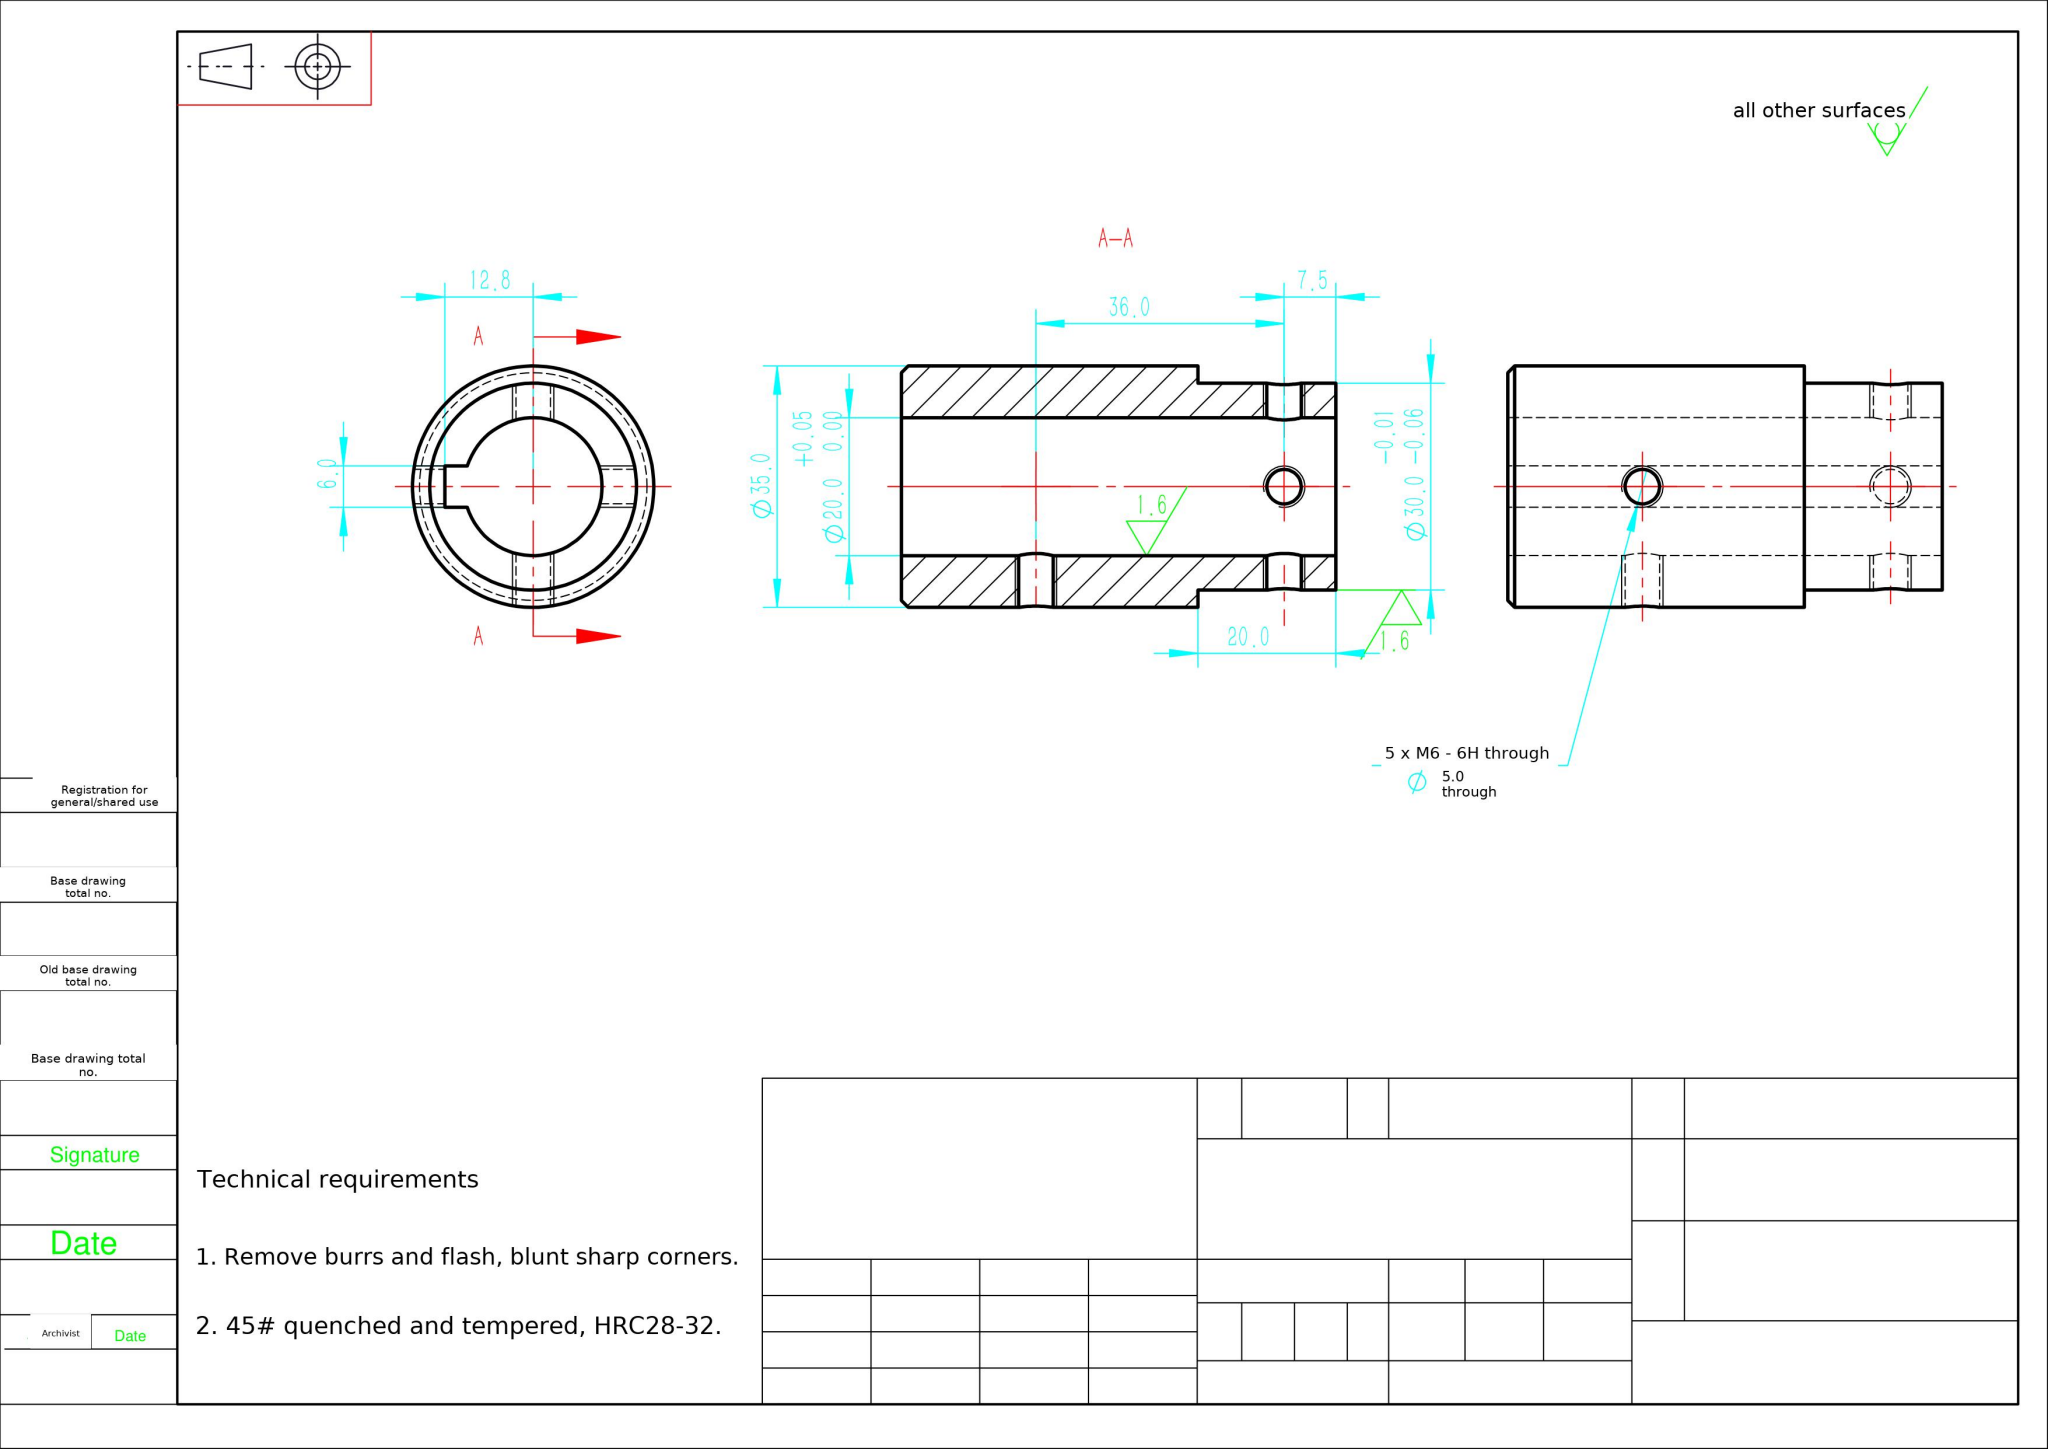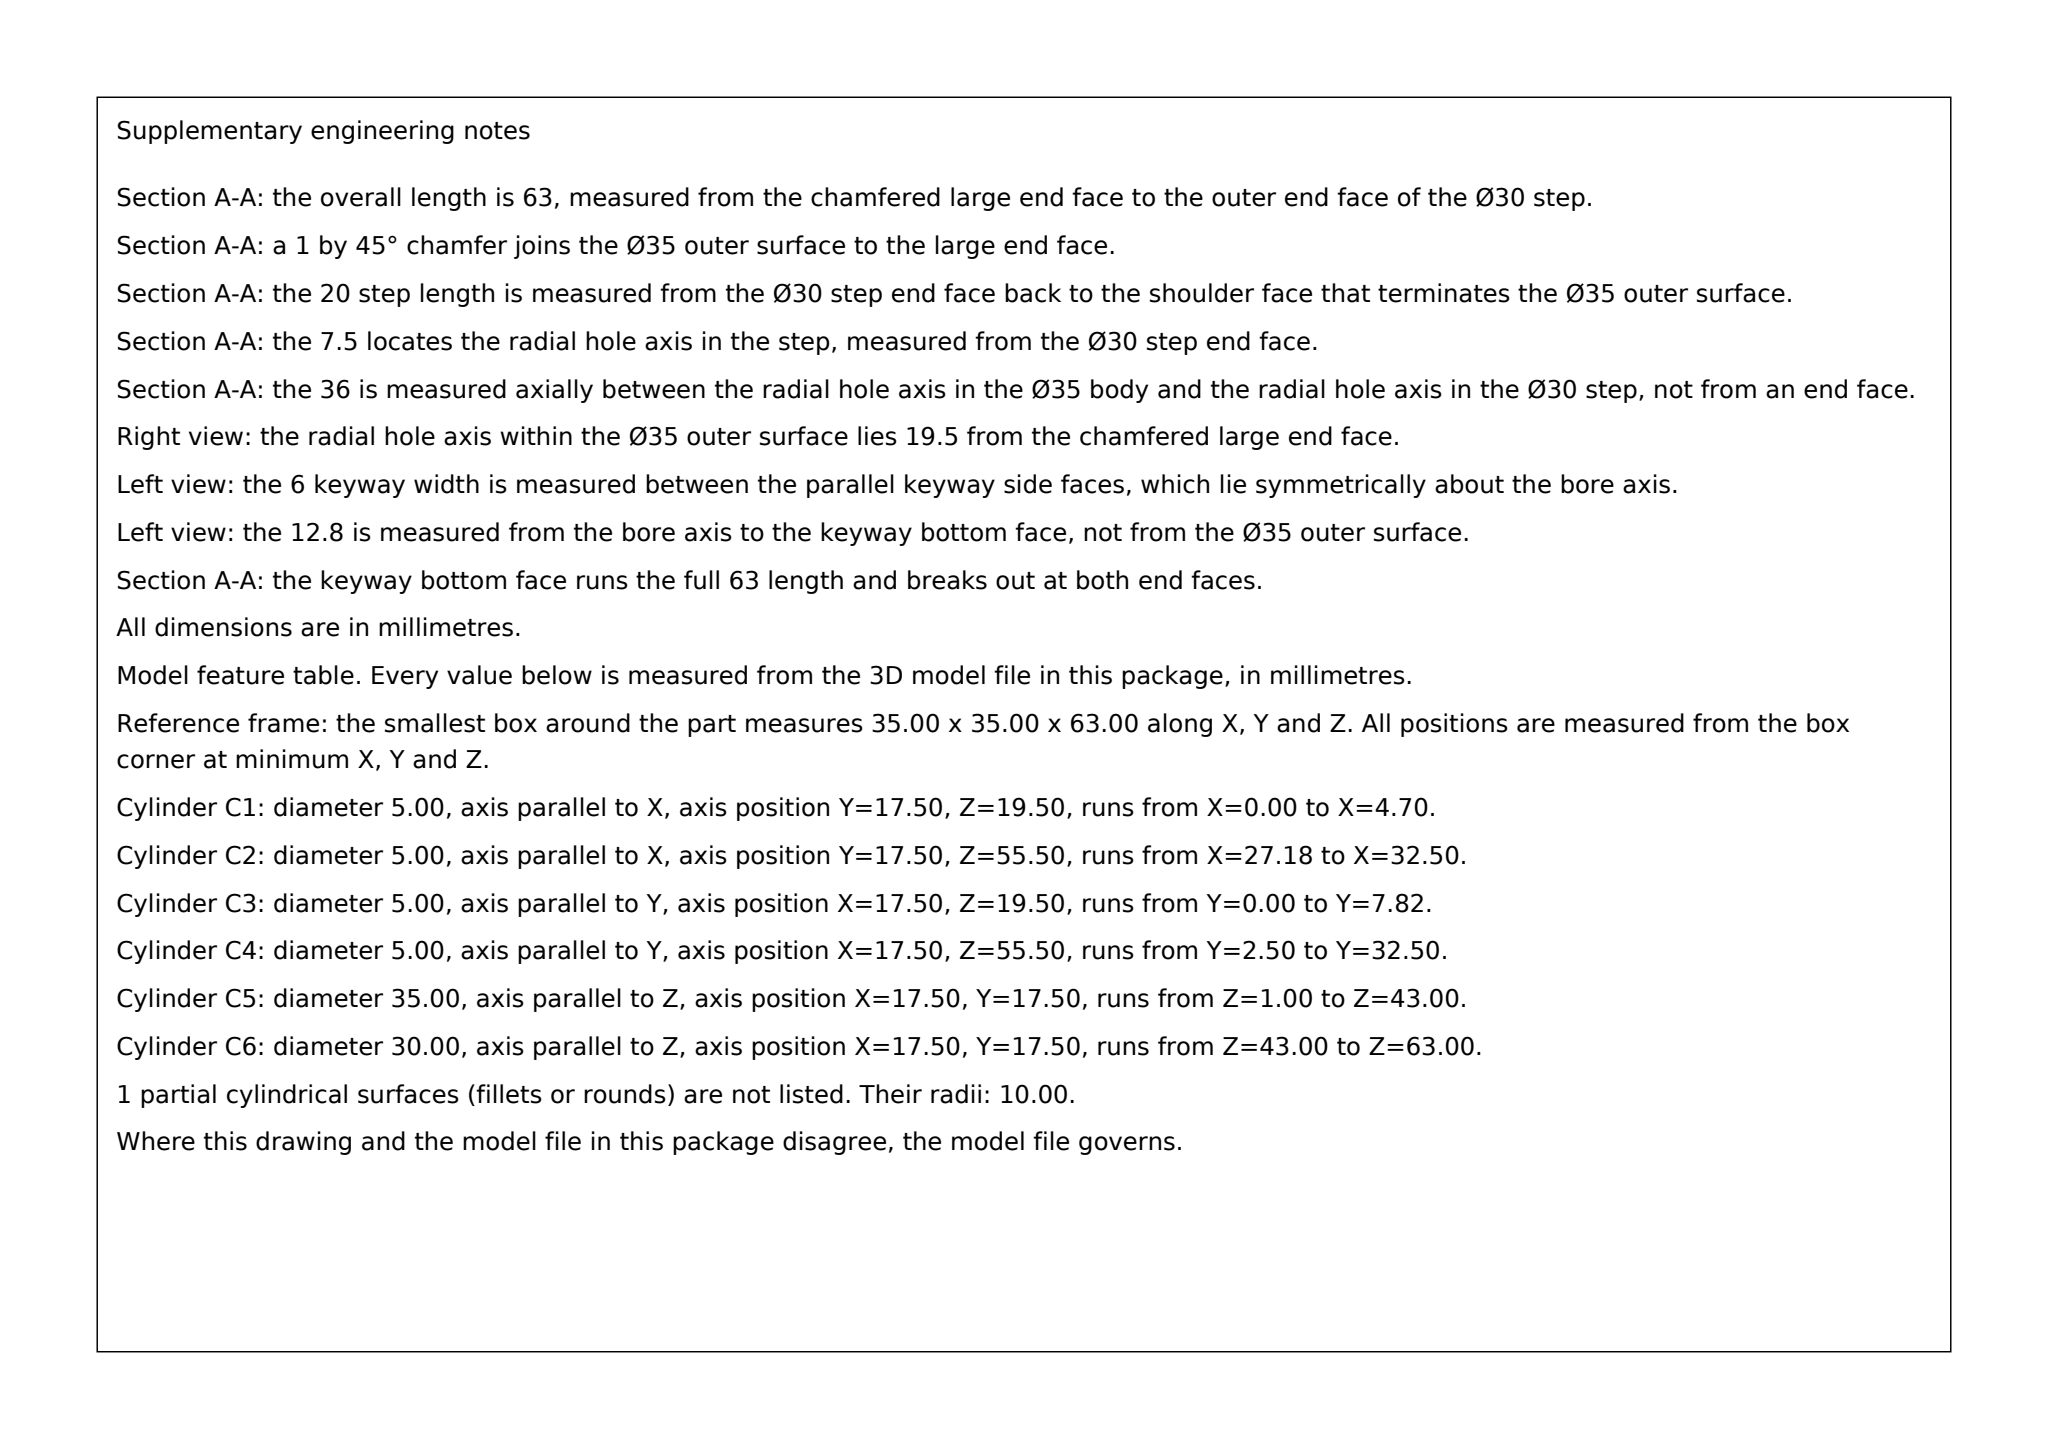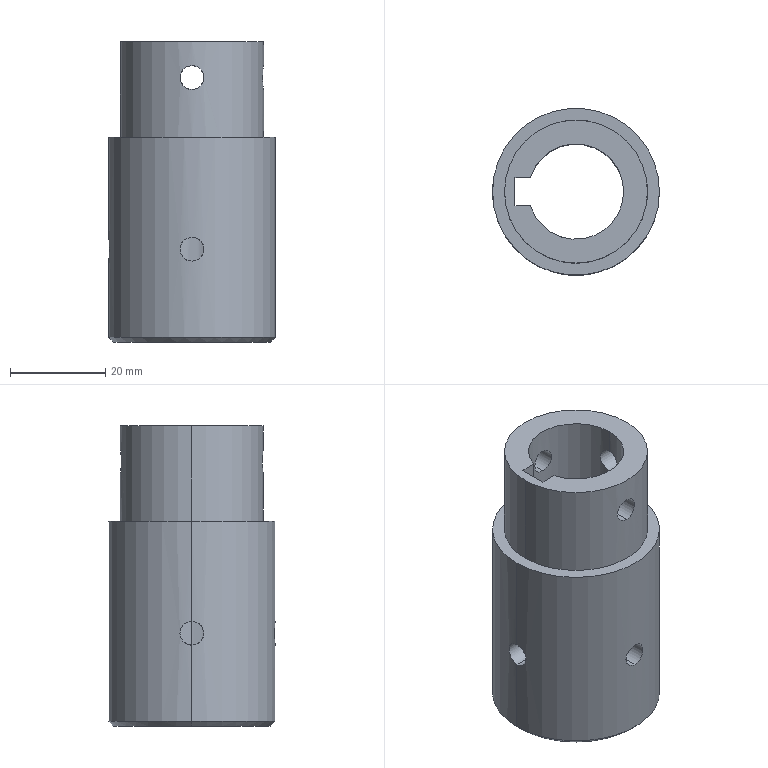Part | SolidWorks | mm | 1 solid | 24 faces | box 35 x 35 x 63 mm | volume 34011 mm3 | cylinder 16 | plane 6 | cone 2 | commonest cylinder face diameters 5 x10 30 x2 20 x2 35 x2
Drawing notes:
M6 HOLE 19.5 FM LH END ON KEYWAY CL, BREAKS INTO KEYWAY | from the solid: Ø5 cyl axis x at y=17.5, z=19.5, len 4.7 ending at keyway floor plane x=4.7 (keyway y 14.5/20.5)
M6 HOLE 19.5 FM LH END AT 90 DEG TO KEYWAY CL, 1 SIDE ONLY | from the solid: Ø5 cyl axis y at x=17.5, z=19.5, len 7.82 (Ø35 wall), single hole
2X M6 IN Ø30 BOSS 7.5 FM RH END AT 90 & 270 DEG TO KEYWAY CL | from the solid: Ø5 cyl axis y at x=17.5, z=55.5, len 5.32, count 4 faces = diametral pair in Ø30 boss (z 43-63)
M6 IN Ø30 BOSS 7.5 FM RH END IN KEYWAY CL PLANE, 90 DEG FM PAIR | from the solid: Ø5 cyl axis x at y=17.5, z=55.5, len 5.32, perpendicular to the y-axis pair at same station
5X M6 HOLES NOT EQSP - SEE ANGULAR NOTES, AXIAL 19.5 & 55.5 FM LH END | from the solid: hole stations z=19.5 and z=55.5 only; 36.0 between stations, 7.5 fm RH end
build123d program:
from build123d import *

# Parameters (mm, degrees)
SKETCH1_R           = 17.5
BOSS_EXTRUDE1_DEPTH = 63
CHAMFER1_SIZE       = 1
SKETCH2_W           = 2.5
SKETCH2_H           = 17.5
SKETCH4_W           = 2.5
SKETCH4_H           = 17.5
SKETCH6_R           = 17.5
SKETCH6_R_2         = 15
CUT_EXTRUDE1_DEPTH  = 20
M6_TAPPED_HOLE3_D   = 5
SKETCH9_W           = 2.5
SKETCH9_H           = 17.5


with BuildPart() as part:
    # Sketch1 → Boss-Extrude1 (new body)
    with BuildSketch(Plane.XY.offset(-27)):
        Circle(SKETCH1_R)
        with BuildLine():
            Line((-12.8, -3), (-9.539, -3))
            ThreePointArc((-9.539, -3), (10, 0), (-9.539, 3))
            Line((-9.539, 3), (-12.8, 3))
            Line((-12.8, 3), (-12.8, -3))
        make_face(mode=Mode.SUBTRACT)
    extrude(amount=-BOSS_EXTRUDE1_DEPTH)

    # Chamfer1
    chamfer1_edges = [part.edges().sort_by_distance(p)[0] for p in [
        (-17.5, 0, -27),
        (-17.5, 0, -90),
    ]]
    chamfer(chamfer1_edges, length=CHAMFER1_SIZE)

    # Sketch2 → M6 Tapped Hole1 (revolve, cut)
    with BuildSketch(Plane(origin=(0, 0, -34.5), x_dir=(0, 0, 1), z_dir=(0, 1, 0))):
        with Locations((1.25, 8.75)):
            Rectangle(SKETCH2_W, SKETCH2_H)
    revolve(axis=Axis((-6.35, 0, -34.5), (1, 0, 0)), mode=Mode.SUBTRACT)

    # Sketch4 → M6 Tapped Hole2 (revolve, cut)
    with BuildSketch(Plane(origin=(0, 0, -70.5), x_dir=(0, 0, 1), z_dir=(1, 0, 0))):
        with Locations((1.25, 8.75)):
            Rectangle(SKETCH4_W, SKETCH4_H)
    revolve(axis=Axis((0, 6.35, -70.5), (0, -1, 0)), mode=Mode.SUBTRACT)

    # Sketch6 → Cut-Extrude1 (cut)
    with BuildSketch(Plane.XY.offset(-27)):
        Circle(SKETCH6_R)
        Circle(SKETCH6_R_2, mode=Mode.SUBTRACT)
    extrude(amount=-CUT_EXTRUDE1_DEPTH, mode=Mode.SUBTRACT)

    # M6 Tapped Hole3 (through all)
    with Locations(Plane(origin=(0, -15, 0), x_dir=(-1, 0, 0), z_dir=(0, -1, 0))):
        with Locations((0, 34.5)):
            Hole(M6_TAPPED_HOLE3_D / 2)

    # Sketch9 → M6 Tapped Hole4 (revolve, cut)
    with BuildSketch(Plane(origin=(0, 0, -70.5), x_dir=(0, 0, -1), z_dir=(0, 1, 0))):
        with Locations((1.25, 8.75)):
            Rectangle(SKETCH9_W, SKETCH9_H)
    revolve(axis=Axis((6.35, 0, -70.5), (-1, 0, 0)), mode=Mode.SUBTRACT)


solid = part.part